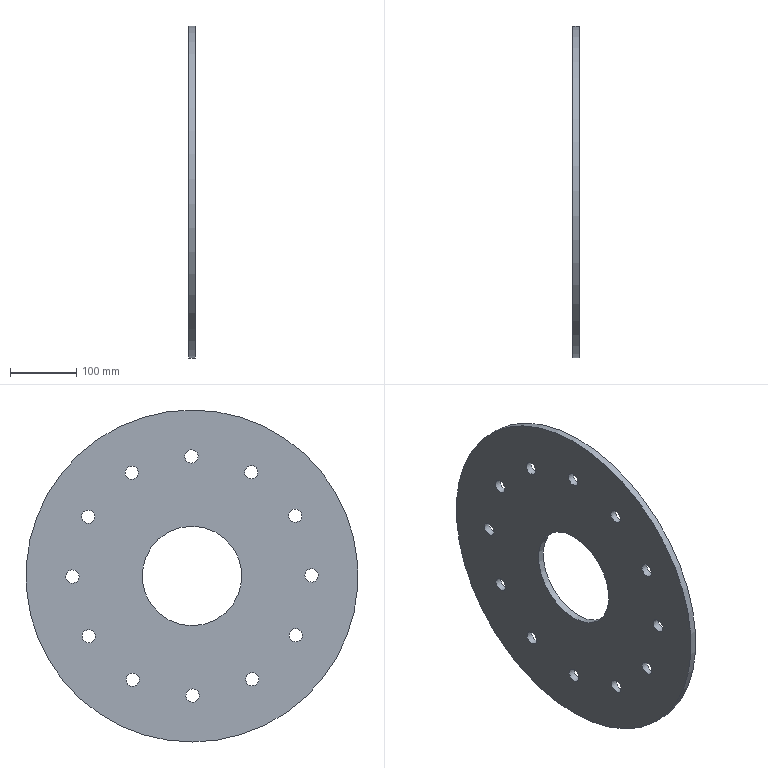Component | NX | BRAKE_PAD | 1 solid | 16 faces | volume 1749082 mm3 | cylinder 14 | plane 2 | commonest cylinder face diameters 20 x12 500 x1 150 x1